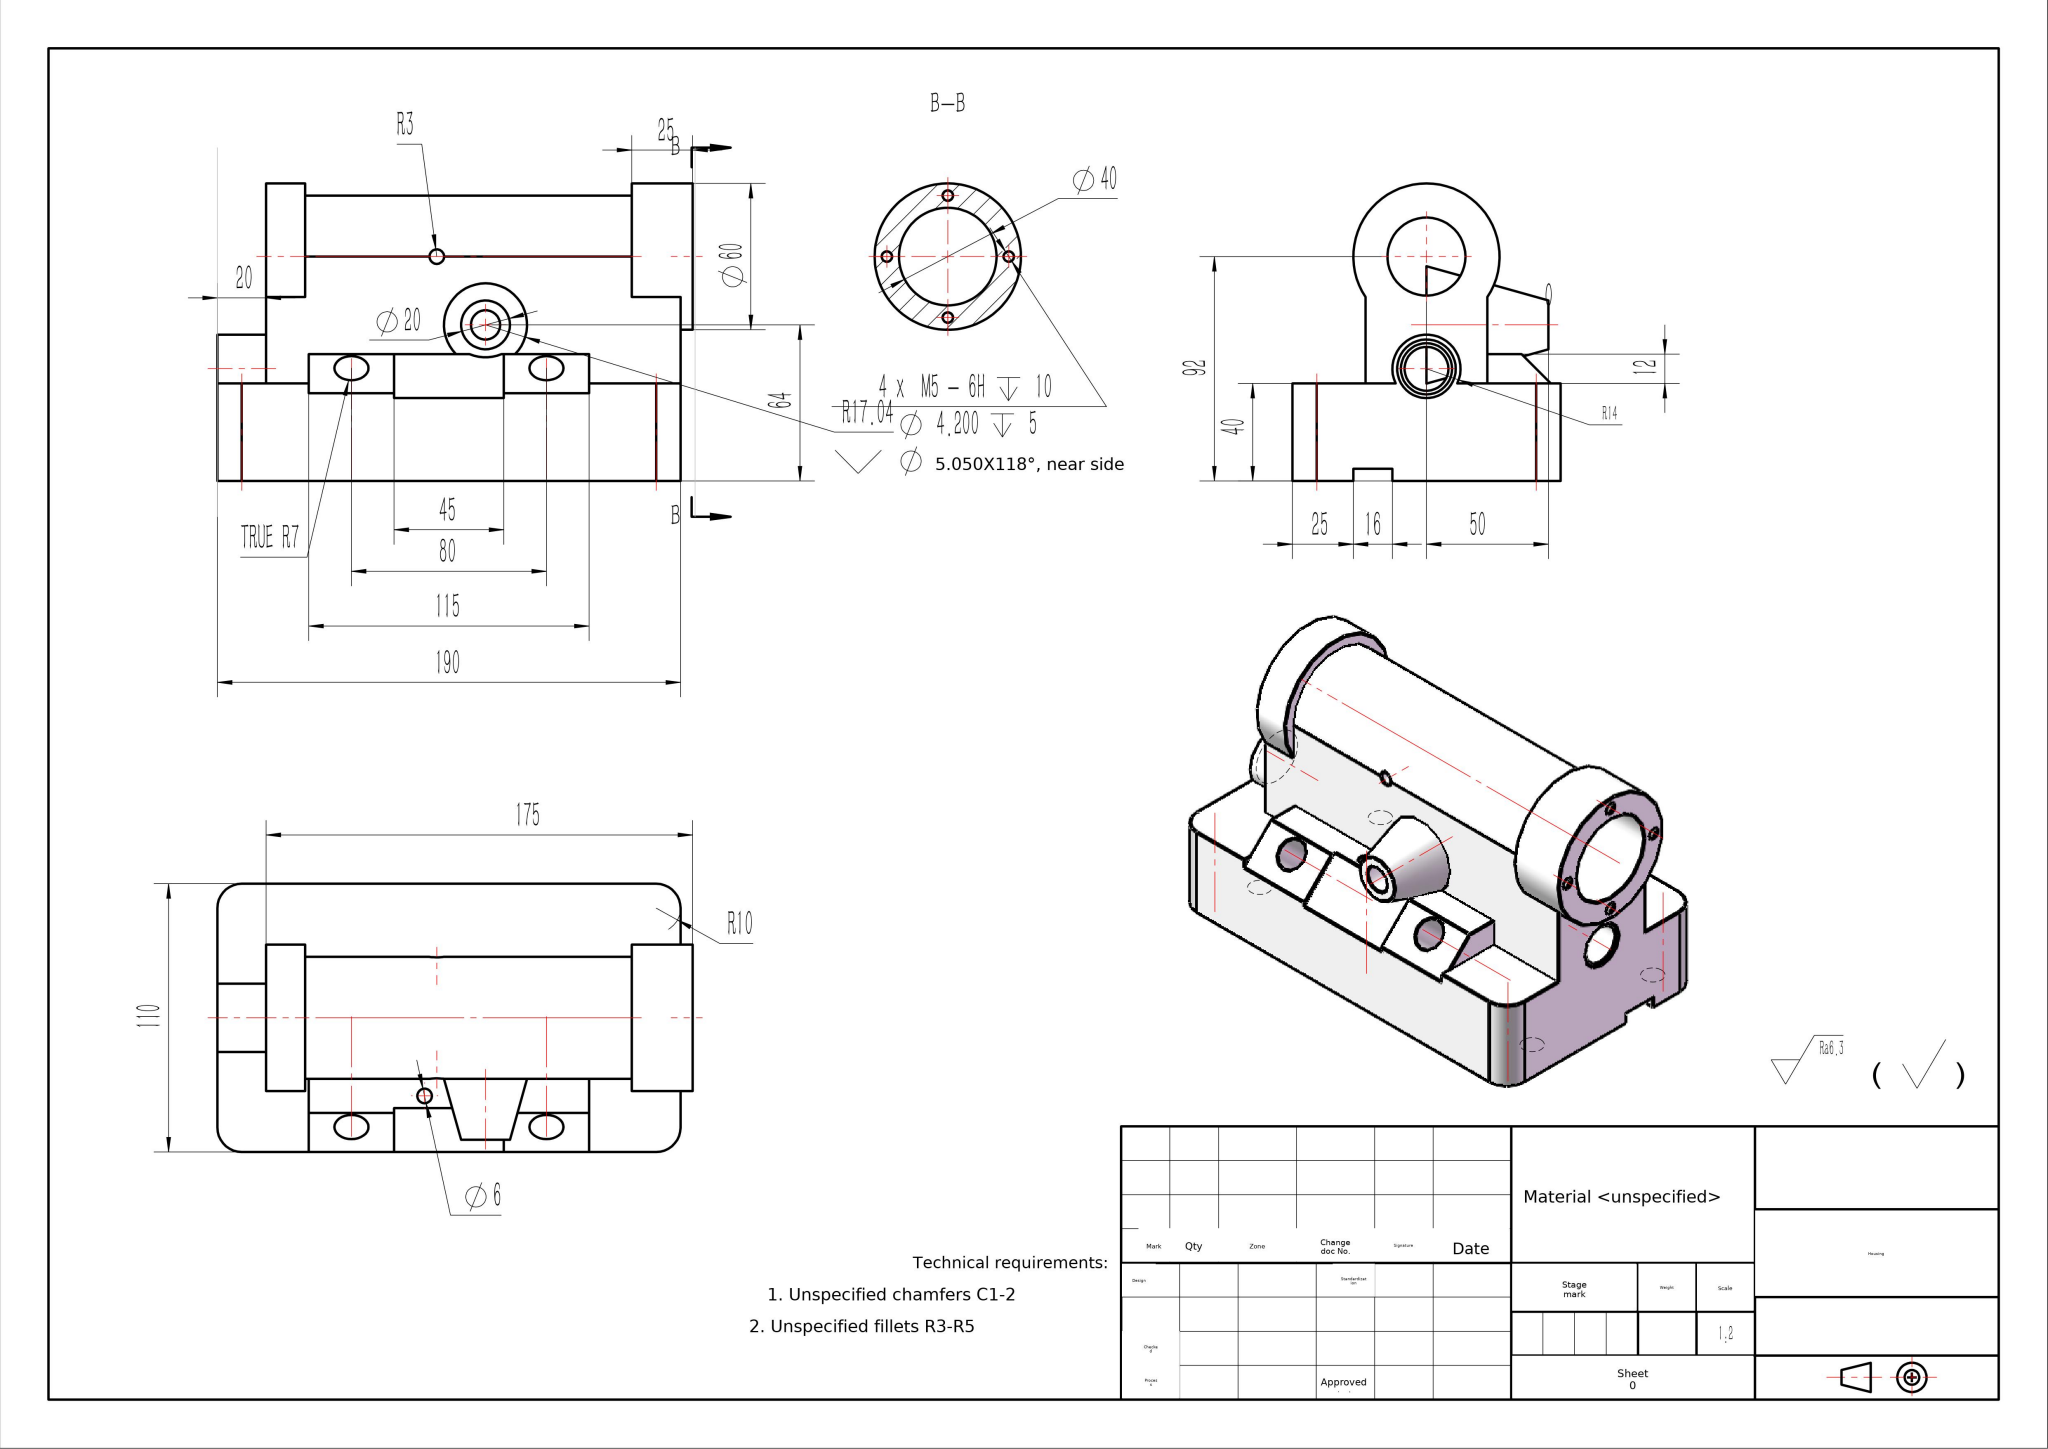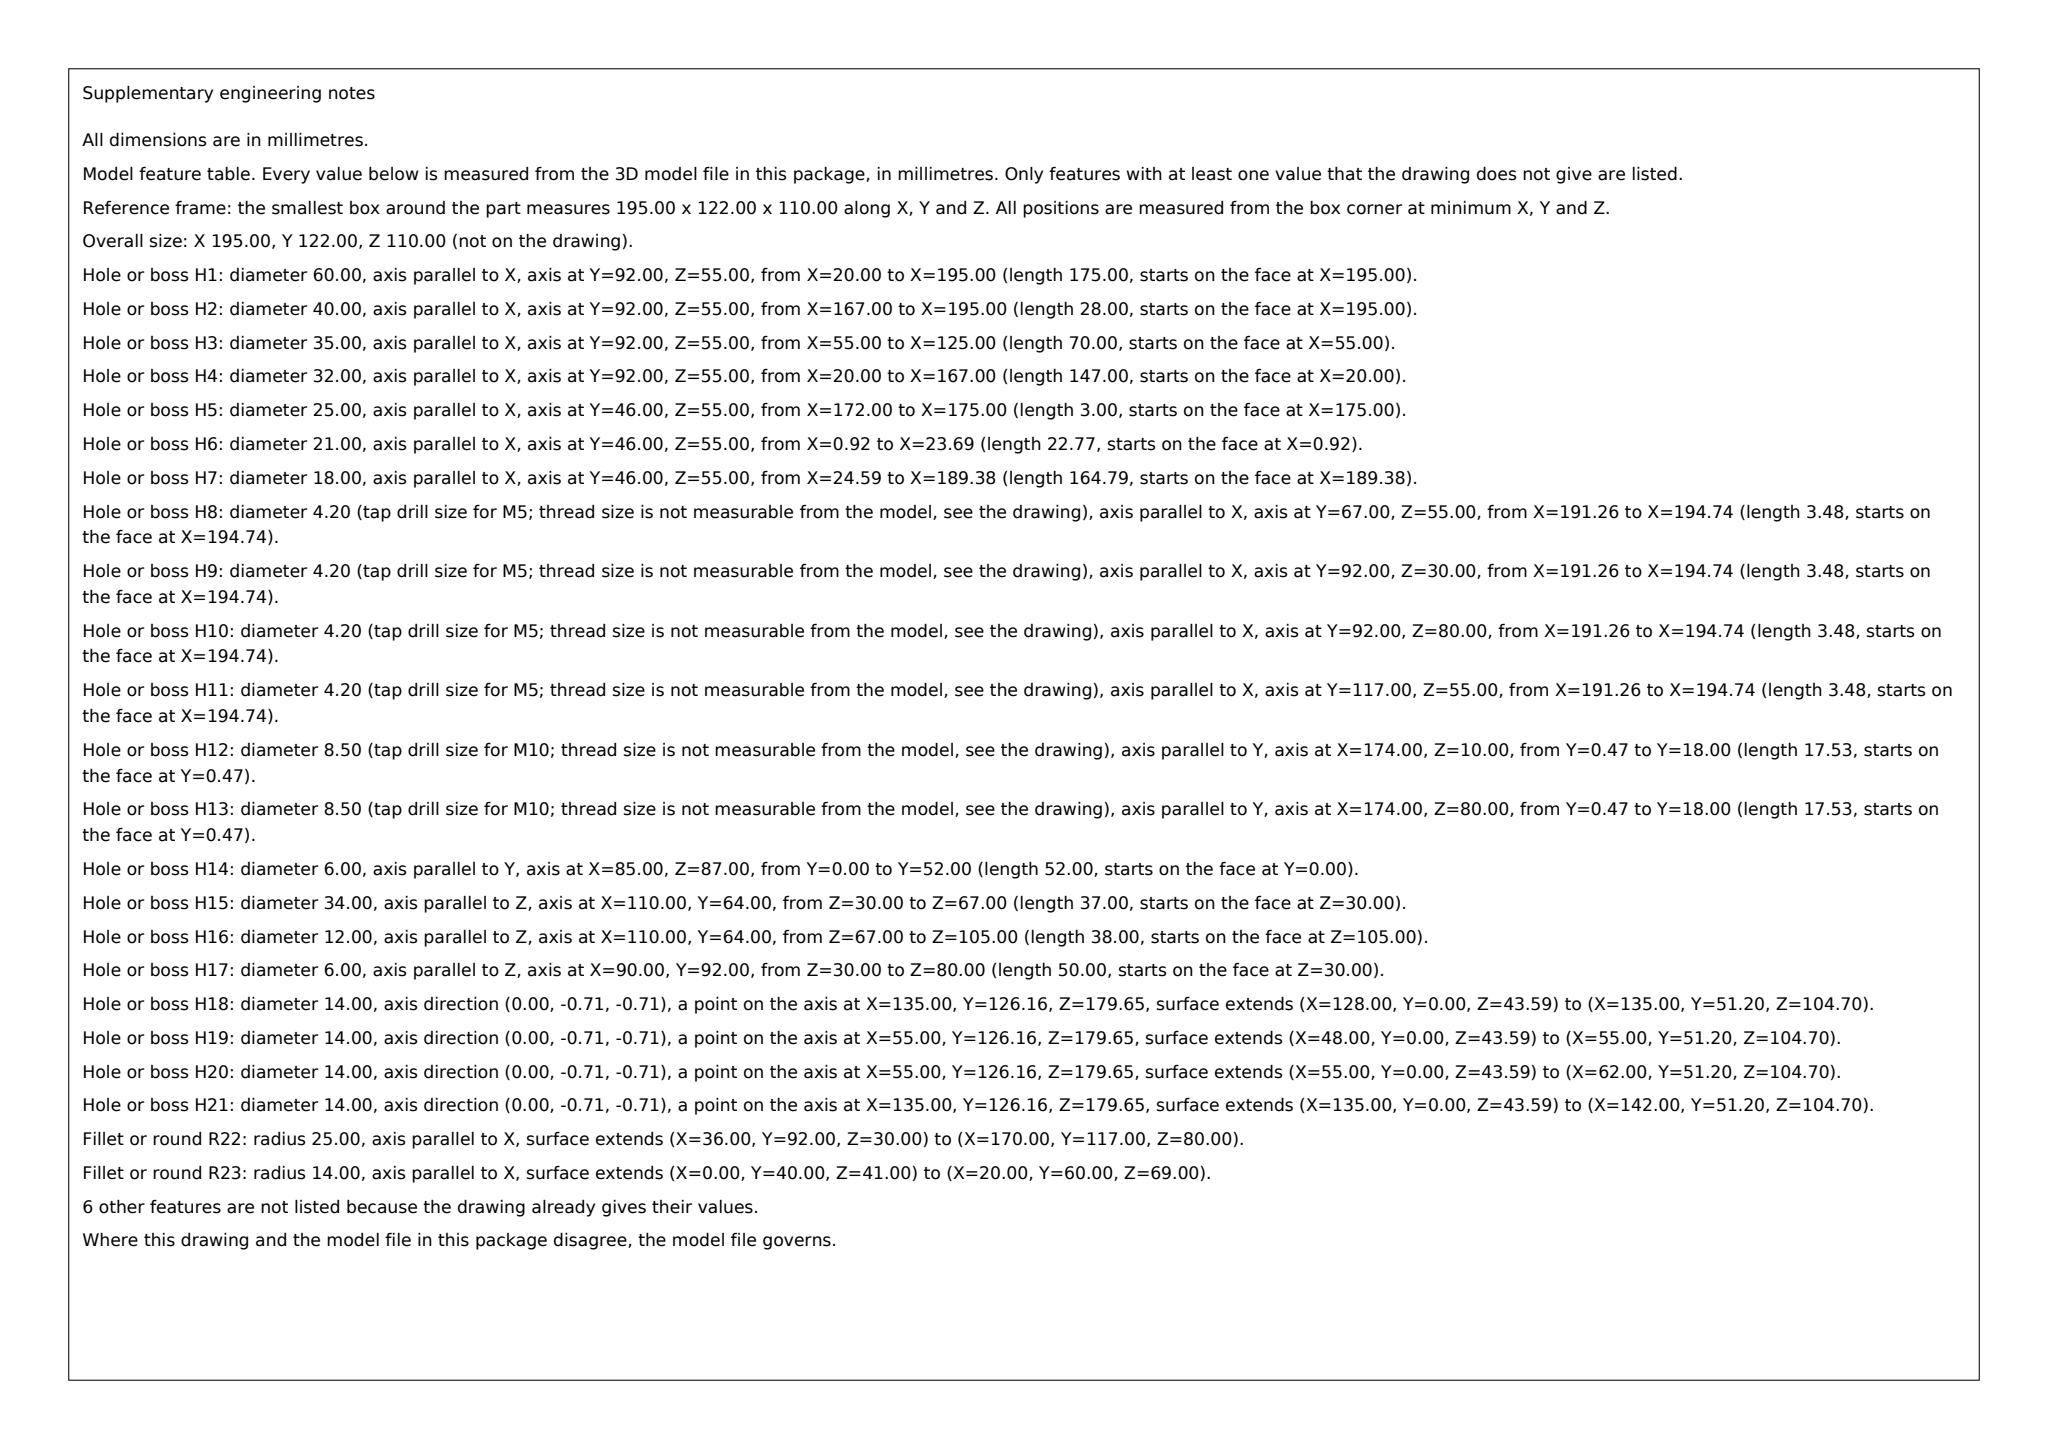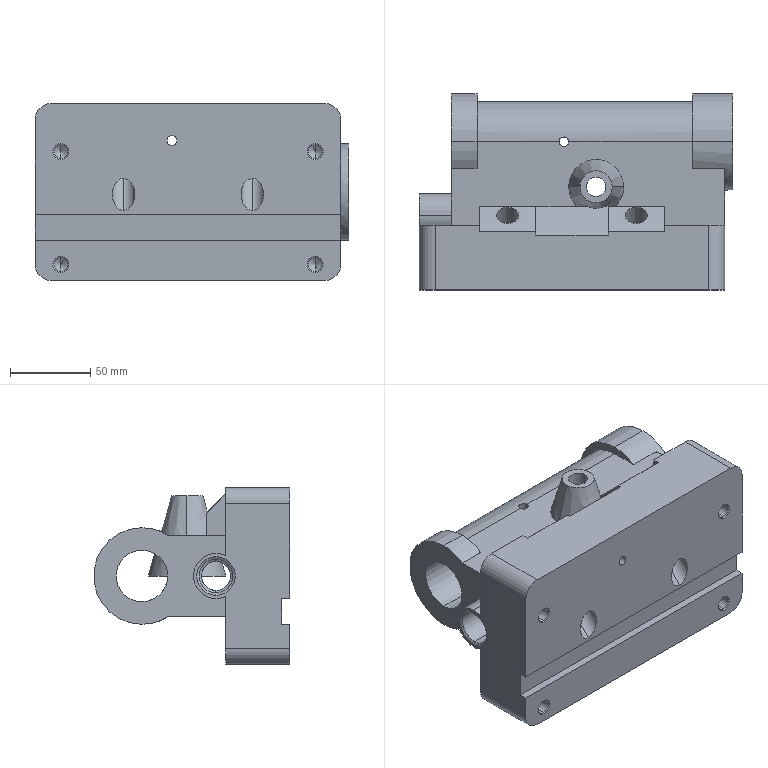Part | SolidWorks | mm | 1 solid | 139 faces | box 195 x 122 x 110 mm | volume 1237088 mm3 | cylinder 59 | cone 42 | plane 38 | commonest cylinder face diameters 8.5 x8 4.2 x8 6 x6 60 x5 14 x4 18 x4 32 x4 20 x4